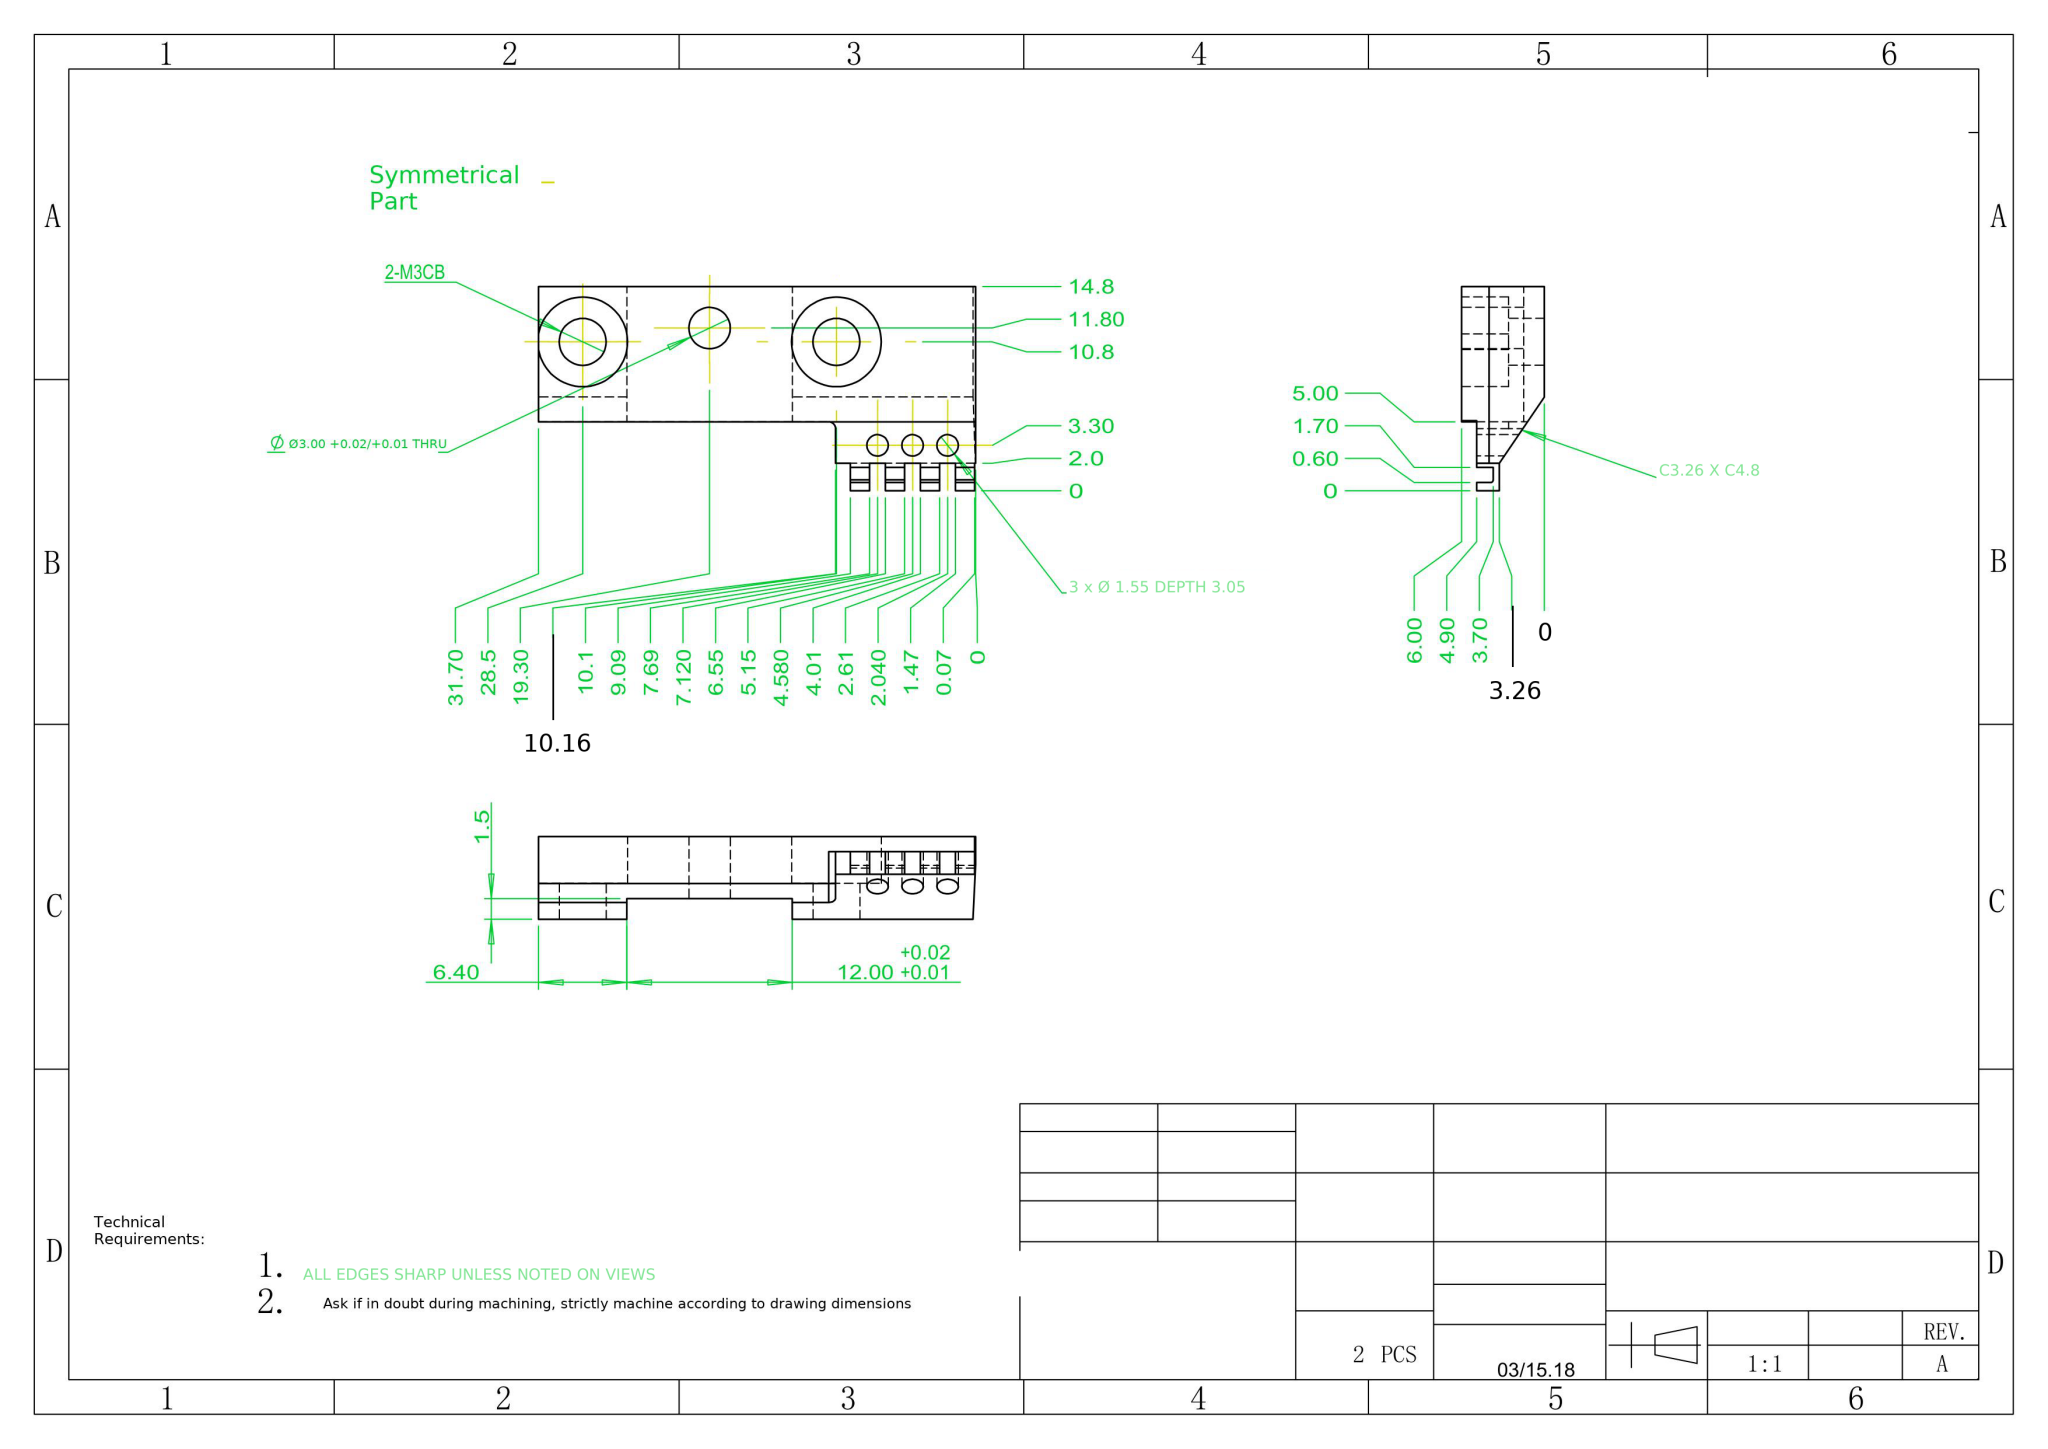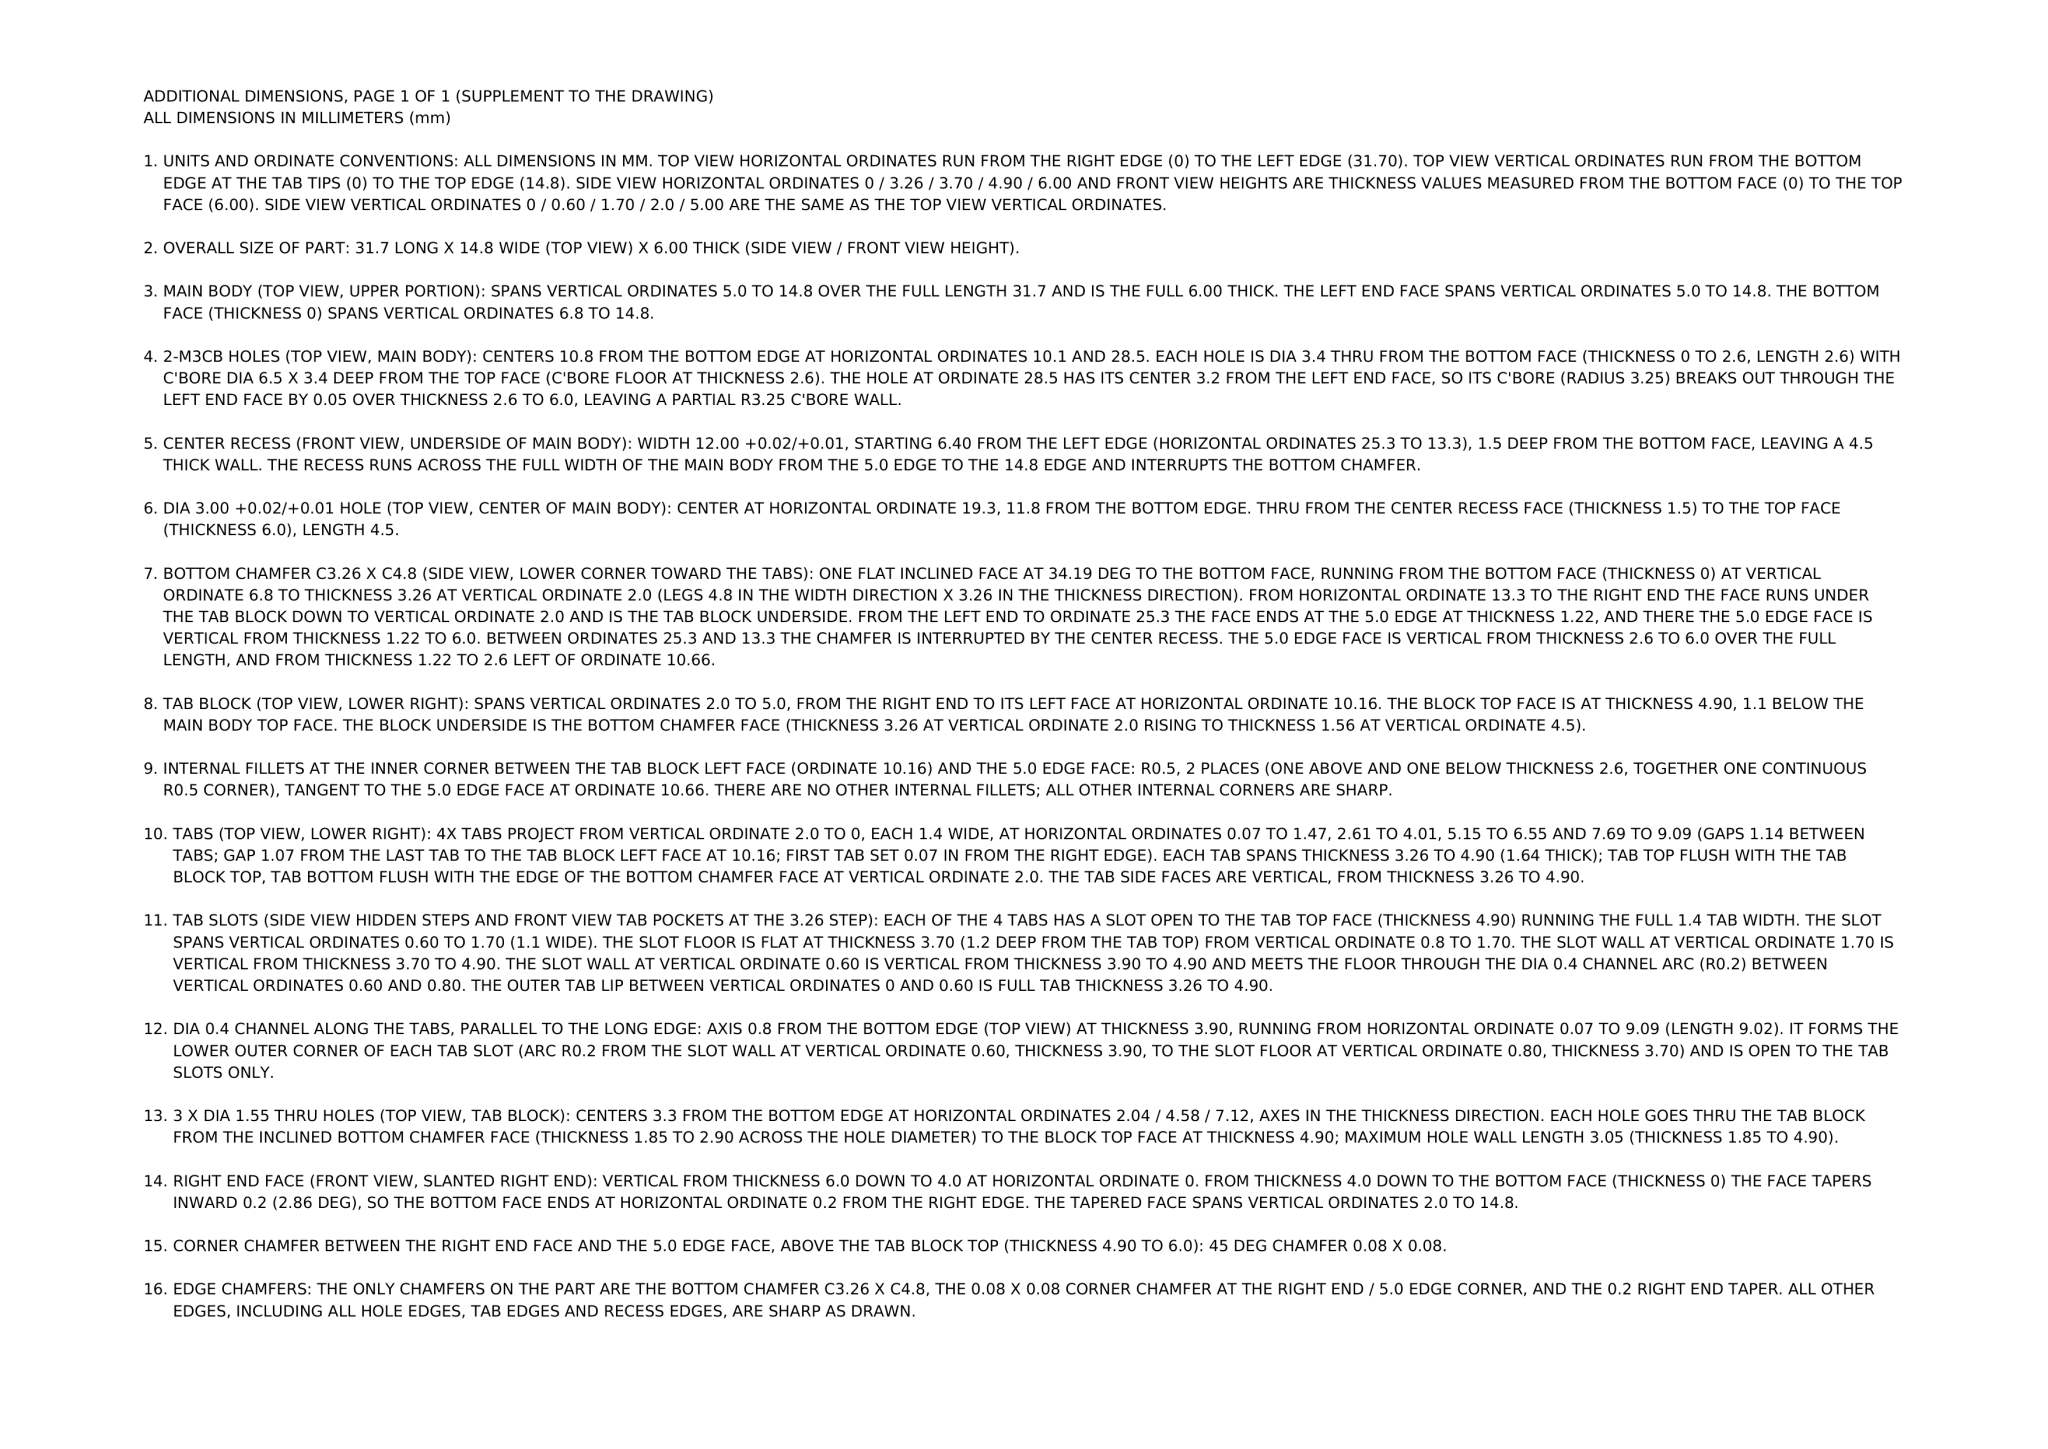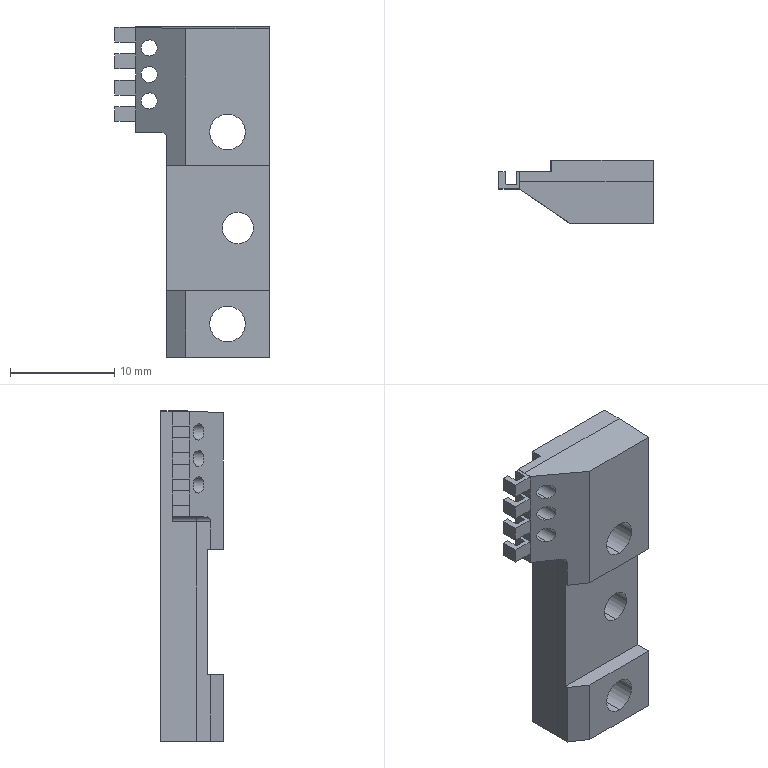Part | NX | mm | 1 solid | 78 faces | box 14.8 x 6 x 31.7 mm | volume 1435 mm3 | plane 56 | cylinder 22 | commonest cylinder face diameters 1.55 x6 6.5 x4 3.4 x4 0.4 x4 3 x2 1 x2